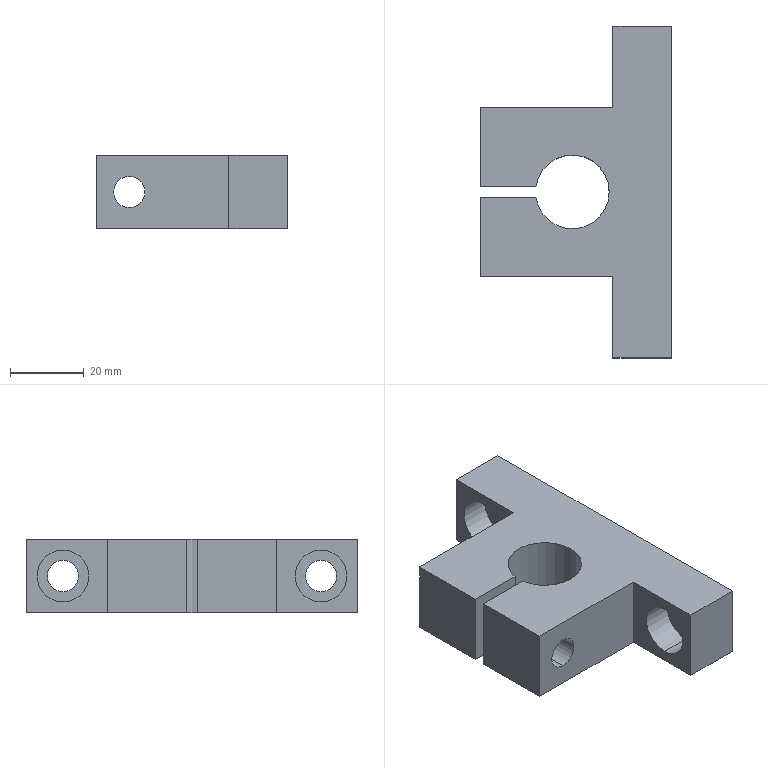Component | SolidWorks | FixedSeat-1 | 1 solid | 31 faces | box 52 x 90 x 20 mm | volume 47991 mm3 | plane 16 | cylinder 15 | commonest cylinder face diameters 8.5 x8 14 x6 20 x1
STEP:
#1=CARTESIAN_POINT('',(-0.4331,19.528,-13.76));
#2=VERTEX_POINT('',#1);
#3=CARTESIAN_POINT('',(-0.4331,19.528,-13.209));
#4=VERTEX_POINT('',#3);
#5=CARTESIAN_POINT('',(-0.4331,19.528,-13.484));
#6=DIRECTION('',(-1.,0.,0.));
#7=DIRECTION('',(0.,0.,1.));
#8=AXIS2_PLACEMENT_3D('',#5,#6,#7);
#9=CIRCLE('',#8,0.2756);
#10=EDGE_CURVE('',#2,#4,#9,.T.);
#11=ORIENTED_EDGE('',*,*,#10,.F.);
#12=CARTESIAN_POINT('',(-0.748,19.528,-13.76));
#13=VERTEX_POINT('',#12);
#14=CARTESIAN_POINT('',(-0.748,19.528,-13.76));
#15=DIRECTION('',(-1.,0.,0.));
#16=VECTOR('',#15,39.37);
#17=LINE('',#14,#16);
#18=EDGE_CURVE('',#2,#13,#17,.T.);
#19=ORIENTED_EDGE('',*,*,#18,.T.);
#20=CARTESIAN_POINT('',(-0.748,19.528,-13.209));
#21=VERTEX_POINT('',#20);
#22=CARTESIAN_POINT('',(-0.748,19.528,-13.484));
#23=DIRECTION('',(-1.,0.,0.));
#24=DIRECTION('',(0.,0.,1.));
#25=AXIS2_PLACEMENT_3D('',#22,#23,#24);
#26=CIRCLE('',#25,0.2756);
#27=EDGE_CURVE('',#13,#21,#26,.T.);
#28=ORIENTED_EDGE('',*,*,#27,.T.);
#29=CARTESIAN_POINT('',(-0.748,19.528,-13.209));
#30=DIRECTION('',(-1.,0.,0.));
#31=VECTOR('',#30,39.37);
#32=LINE('',#29,#31);
#33=EDGE_CURVE('',#4,#21,#32,.T.);
#34=ORIENTED_EDGE('',*,*,#33,.F.);
#35=EDGE_LOOP('',(#11,#19,#28,#34));
#36=FACE_OUTER_BOUND('',#35,.T.);
#37=CARTESIAN_POINT('',(-0.748,19.528,-13.484));
#38=DIRECTION('',(-1.,0.,0.));
#39=DIRECTION('',(0.,0.,1.));
#40=AXIS2_PLACEMENT_3D('',#37,#38,#39);
#41=CYLINDRICAL_SURFACE('',#40,0.2756);
#42=ADVANCED_FACE('',(#36),#41,.F.);
#43=CARTESIAN_POINT('',(-0.1181,19.528,-13.652));
#44=VERTEX_POINT('',#43);
#45=CARTESIAN_POINT('',(-0.1181,19.528,-13.317));
#46=VERTEX_POINT('',#45);
#47=CARTESIAN_POINT('',(-0.1181,19.528,-13.484));
#48=DIRECTION('',(-1.,0.,0.));
#49=DIRECTION('',(0.,0.,1.));
#50=AXIS2_PLACEMENT_3D('',#47,#48,#49);
#51=CIRCLE('',#50,0.1673);
#52=EDGE_CURVE('',#44,#46,#51,.T.);
#53=ORIENTED_EDGE('',*,*,#52,.F.);
#54=CARTESIAN_POINT('',(-0.4331,19.528,-13.652));
#55=VERTEX_POINT('',#54);
#56=CARTESIAN_POINT('',(-0.748,19.528,-13.652));
#57=DIRECTION('',(-1.,0.,0.));
#58=VECTOR('',#57,39.37);
#59=LINE('',#56,#58);
#60=EDGE_CURVE('',#44,#55,#59,.T.);
#61=ORIENTED_EDGE('',*,*,#60,.T.);
#62=CARTESIAN_POINT('',(-0.4331,19.528,-13.317));
#63=VERTEX_POINT('',#62);
#64=CARTESIAN_POINT('',(-0.4331,19.528,-13.484));
#65=DIRECTION('',(-1.,0.,0.));
#66=DIRECTION('',(0.,0.,1.));
#67=AXIS2_PLACEMENT_3D('',#64,#65,#66);
#68=CIRCLE('',#67,0.1673);
#69=EDGE_CURVE('',#55,#63,#68,.T.);
#70=ORIENTED_EDGE('',*,*,#69,.T.);
#71=CARTESIAN_POINT('',(-0.748,19.528,-13.317));
#72=DIRECTION('',(-1.,0.,0.));
#73=VECTOR('',#72,39.37);
#74=LINE('',#71,#73);
#75=EDGE_CURVE('',#46,#63,#74,.T.);
#76=ORIENTED_EDGE('',*,*,#75,.F.);
#77=EDGE_LOOP('',(#53,#61,#70,#76));
#78=FACE_OUTER_BOUND('',#77,.T.);
#79=CARTESIAN_POINT('',(-0.748,19.528,-13.484));
#80=DIRECTION('',(-1.,0.,0.));
#81=DIRECTION('',(0.,0.,1.));
#82=AXIS2_PLACEMENT_3D('',#79,#80,#81);
#83=CYLINDRICAL_SURFACE('',#82,0.1673);
#84=ADVANCED_FACE('',(#78),#83,.F.);
#85=CARTESIAN_POINT('',(-0.4331,16.772,-13.76));
#86=VERTEX_POINT('',#85);
#87=CARTESIAN_POINT('',(-0.4331,16.772,-13.209));
#88=VERTEX_POINT('',#87);
#89=CARTESIAN_POINT('',(-0.4331,16.772,-13.484));
#90=DIRECTION('',(-1.,0.,0.));
#91=DIRECTION('',(0.,0.,1.));
#92=AXIS2_PLACEMENT_3D('',#89,#90,#91);
#93=CIRCLE('',#92,0.2756);
#94=EDGE_CURVE('',#86,#88,#93,.T.);
#95=ORIENTED_EDGE('',*,*,#94,.F.);
#96=CARTESIAN_POINT('',(-0.748,16.772,-13.76));
#97=VERTEX_POINT('',#96);
#98=CARTESIAN_POINT('',(-0.748,16.772,-13.76));
#99=DIRECTION('',(-1.,0.,0.));
#100=VECTOR('',#99,39.37);
#101=LINE('',#98,#100);
#102=EDGE_CURVE('',#86,#97,#101,.T.);
#103=ORIENTED_EDGE('',*,*,#102,.T.);
#104=CARTESIAN_POINT('',(-0.748,16.772,-13.209));
#105=VERTEX_POINT('',#104);
#106=CARTESIAN_POINT('',(-0.748,16.772,-13.484));
#107=DIRECTION('',(-1.,0.,0.));
#108=DIRECTION('',(0.,0.,1.));
#109=AXIS2_PLACEMENT_3D('',#106,#107,#108);
#110=CIRCLE('',#109,0.2756);
#111=EDGE_CURVE('',#97,#105,#110,.T.);
#112=ORIENTED_EDGE('',*,*,#111,.T.);
#113=CARTESIAN_POINT('',(-0.748,16.772,-13.209));
#114=DIRECTION('',(-1.,0.,0.));
#115=VECTOR('',#114,39.37);
#116=LINE('',#113,#115);
#117=EDGE_CURVE('',#88,#105,#116,.T.);
#118=ORIENTED_EDGE('',*,*,#117,.F.);
#119=EDGE_LOOP('',(#95,#103,#112,#118));
#120=FACE_OUTER_BOUND('',#119,.T.);
#121=CARTESIAN_POINT('',(-0.748,16.772,-13.484));
#122=DIRECTION('',(-1.,0.,0.));
#123=DIRECTION('',(0.,0.,1.));
#124=AXIS2_PLACEMENT_3D('',#121,#122,#123);
#125=CYLINDRICAL_SURFACE('',#124,0.2756);
#126=ADVANCED_FACE('',(#120),#125,.F.);
#127=CARTESIAN_POINT('',(-0.1181,16.772,-13.652));
#128=VERTEX_POINT('',#127);
#129=CARTESIAN_POINT('',(-0.1181,16.772,-13.317));
#130=VERTEX_POINT('',#129);
#131=CARTESIAN_POINT('',(-0.1181,16.772,-13.484));
#132=DIRECTION('',(-1.,0.,0.));
#133=DIRECTION('',(0.,0.,1.));
#134=AXIS2_PLACEMENT_3D('',#131,#132,#133);
#135=CIRCLE('',#134,0.1673);
#136=EDGE_CURVE('',#128,#130,#135,.T.);
#137=ORIENTED_EDGE('',*,*,#136,.F.);
#138=CARTESIAN_POINT('',(-0.4331,16.772,-13.652));
#139=VERTEX_POINT('',#138);
#140=CARTESIAN_POINT('',(-0.748,16.772,-13.652));
#141=DIRECTION('',(-1.,0.,0.));
#142=VECTOR('',#141,39.37);
#143=LINE('',#140,#142);
#144=EDGE_CURVE('',#128,#139,#143,.T.);
#145=ORIENTED_EDGE('',*,*,#144,.T.);
#146=CARTESIAN_POINT('',(-0.4331,16.772,-13.317));
#147=VERTEX_POINT('',#146);
#148=CARTESIAN_POINT('',(-0.4331,16.772,-13.484));
#149=DIRECTION('',(-1.,0.,0.));
#150=DIRECTION('',(0.,0.,1.));
#151=AXIS2_PLACEMENT_3D('',#148,#149,#150);
#152=CIRCLE('',#151,0.1673);
#153=EDGE_CURVE('',#139,#147,#152,.T.);
#154=ORIENTED_EDGE('',*,*,#153,.T.);
#155=CARTESIAN_POINT('',(-0.748,16.772,-13.317));
#156=DIRECTION('',(-1.,0.,0.));
#157=VECTOR('',#156,39.37);
#158=LINE('',#155,#157);
#159=EDGE_CURVE('',#130,#147,#158,.T.);
#160=ORIENTED_EDGE('',*,*,#159,.F.);
#161=EDGE_LOOP('',(#137,#145,#154,#160));
#162=FACE_OUTER_BOUND('',#161,.T.);
#163=CARTESIAN_POINT('',(-0.748,16.772,-13.484));
#164=DIRECTION('',(-1.,0.,0.));
#165=DIRECTION('',(0.,0.,1.));
#166=AXIS2_PLACEMENT_3D('',#163,#164,#165);
#167=CYLINDRICAL_SURFACE('',#166,0.1673);
#168=ADVANCED_FACE('',(#162),#167,.F.);
#169=CARTESIAN_POINT('',(-1.811,18.677,-13.76));
#170=VERTEX_POINT('',#169);
#171=CARTESIAN_POINT('',(-1.811,18.677,-13.209));
#172=VERTEX_POINT('',#171);
#173=CARTESIAN_POINT('',(-1.811,18.677,-13.484));
#174=DIRECTION('',(0.,1.,0.));
#175=DIRECTION('',(0.,0.,1.));
#176=AXIS2_PLACEMENT_3D('',#173,#174,#175);
#177=CIRCLE('',#176,0.2756);
#178=EDGE_CURVE('',#170,#172,#177,.T.);
#179=ORIENTED_EDGE('',*,*,#178,.F.);
#180=CARTESIAN_POINT('',(-1.811,19.055,-13.76));
#181=VERTEX_POINT('',#180);
#182=CARTESIAN_POINT('',(-1.811,19.055,-13.76));
#183=DIRECTION('',(0.,1.,0.));
#184=VECTOR('',#183,39.37);
#185=LINE('',#182,#184);
#186=EDGE_CURVE('',#170,#181,#185,.T.);
#187=ORIENTED_EDGE('',*,*,#186,.T.);
#188=CARTESIAN_POINT('',(-1.811,19.055,-13.209));
#189=VERTEX_POINT('',#188);
#190=CARTESIAN_POINT('',(-1.811,19.055,-13.484));
#191=DIRECTION('',(0.,1.,0.));
#192=DIRECTION('',(0.,0.,1.));
#193=AXIS2_PLACEMENT_3D('',#190,#191,#192);
#194=CIRCLE('',#193,0.2756);
#195=EDGE_CURVE('',#181,#189,#194,.T.);
#196=ORIENTED_EDGE('',*,*,#195,.T.);
#197=CARTESIAN_POINT('',(-1.811,19.055,-13.209));
#198=DIRECTION('',(0.,1.,0.));
#199=VECTOR('',#198,39.37);
#200=LINE('',#197,#199);
#201=EDGE_CURVE('',#172,#189,#200,.T.);
#202=ORIENTED_EDGE('',*,*,#201,.F.);
#203=EDGE_LOOP('',(#179,#187,#196,#202));
#204=FACE_OUTER_BOUND('',#203,.T.);
#205=CARTESIAN_POINT('',(-1.811,19.055,-13.484));
#206=DIRECTION('',(0.,1.,0.));
#207=DIRECTION('',(0.,0.,1.));
#208=AXIS2_PLACEMENT_3D('',#205,#206,#207);
#209=CYLINDRICAL_SURFACE('',#208,0.2756);
#210=ADVANCED_FACE('',(#204),#209,.F.);
#211=CARTESIAN_POINT('',(-1.811,18.209,-13.652));
#212=VERTEX_POINT('',#211);
#213=CARTESIAN_POINT('',(-1.811,18.209,-13.317));
#214=VERTEX_POINT('',#213);
#215=CARTESIAN_POINT('',(-1.811,18.209,-13.484));
#216=DIRECTION('',(-0.,1.,0.));
#217=DIRECTION('',(-1.,0.,0.));
#218=AXIS2_PLACEMENT_3D('',#215,#216,#217);
#219=CIRCLE('',#218,0.1673);
#220=EDGE_CURVE('',#212,#214,#219,.T.);
#221=ORIENTED_EDGE('',*,*,#220,.F.);
#222=CARTESIAN_POINT('',(-1.811,18.677,-13.652));
#223=VERTEX_POINT('',#222);
#224=CARTESIAN_POINT('',(-1.811,19.055,-13.652));
#225=DIRECTION('',(0.,1.,0.));
#226=VECTOR('',#225,39.37);
#227=LINE('',#224,#226);
#228=EDGE_CURVE('',#212,#223,#227,.T.);
#229=ORIENTED_EDGE('',*,*,#228,.T.);
#230=CARTESIAN_POINT('',(-1.811,18.677,-13.317));
#231=VERTEX_POINT('',#230);
#232=CARTESIAN_POINT('',(-1.811,18.677,-13.484));
#233=DIRECTION('',(0.,1.,0.));
#234=DIRECTION('',(0.,0.,1.));
#235=AXIS2_PLACEMENT_3D('',#232,#233,#234);
#236=CIRCLE('',#235,0.1673);
#237=EDGE_CURVE('',#223,#231,#236,.T.);
#238=ORIENTED_EDGE('',*,*,#237,.T.);
#239=CARTESIAN_POINT('',(-1.811,19.055,-13.317));
#240=DIRECTION('',(0.,1.,0.));
#241=VECTOR('',#240,39.37);
#242=LINE('',#239,#241);
#243=EDGE_CURVE('',#214,#231,#242,.T.);
#244=ORIENTED_EDGE('',*,*,#243,.F.);
#245=EDGE_LOOP('',(#221,#229,#238,#244));
#246=FACE_OUTER_BOUND('',#245,.T.);
#247=CARTESIAN_POINT('',(-1.811,19.055,-13.484));
#248=DIRECTION('',(0.,1.,0.));
#249=DIRECTION('',(0.,0.,1.));
#250=AXIS2_PLACEMENT_3D('',#247,#248,#249);
#251=CYLINDRICAL_SURFACE('',#250,0.1673);
#252=ADVANCED_FACE('',(#246),#251,.F.);
#253=CARTESIAN_POINT('',(-1.811,17.244,-13.652));
#254=VERTEX_POINT('',#253);
#255=CARTESIAN_POINT('',(-1.811,17.244,-13.317));
#256=VERTEX_POINT('',#255);
#257=CARTESIAN_POINT('',(-1.811,17.244,-13.484));
#258=DIRECTION('',(0.,1.,0.));
#259=DIRECTION('',(0.,0.,1.));
#260=AXIS2_PLACEMENT_3D('',#257,#258,#259);
#261=CIRCLE('',#260,0.1673);
#262=EDGE_CURVE('',#254,#256,#261,.T.);
#263=ORIENTED_EDGE('',*,*,#262,.F.);
#264=CARTESIAN_POINT('',(-1.811,18.091,-13.652));
#265=VERTEX_POINT('',#264);
#266=CARTESIAN_POINT('',(-1.811,19.055,-13.652));
#267=DIRECTION('',(0.,1.,0.));
#268=VECTOR('',#267,39.37);
#269=LINE('',#266,#268);
#270=EDGE_CURVE('',#254,#265,#269,.T.);
#271=ORIENTED_EDGE('',*,*,#270,.T.);
#272=CARTESIAN_POINT('',(-1.811,18.091,-13.317));
#273=VERTEX_POINT('',#272);
#274=CARTESIAN_POINT('',(-1.811,18.091,-13.484));
#275=DIRECTION('',(0.,-1.,0.));
#276=DIRECTION('',(1.,0.,0.));
#277=AXIS2_PLACEMENT_3D('',#274,#275,#276);
#278=CIRCLE('',#277,0.1673);
#279=EDGE_CURVE('',#273,#265,#278,.T.);
#280=ORIENTED_EDGE('',*,*,#279,.F.);
#281=CARTESIAN_POINT('',(-1.811,19.055,-13.317));
#282=DIRECTION('',(0.,1.,0.));
#283=VECTOR('',#282,39.37);
#284=LINE('',#281,#283);
#285=EDGE_CURVE('',#256,#273,#284,.T.);
#286=ORIENTED_EDGE('',*,*,#285,.F.);
#287=EDGE_LOOP('',(#263,#271,#280,#286));
#288=FACE_OUTER_BOUND('',#287,.T.);
#289=CARTESIAN_POINT('',(-1.811,19.055,-13.484));
#290=DIRECTION('',(0.,1.,0.));
#291=DIRECTION('',(0.,0.,1.));
#292=AXIS2_PLACEMENT_3D('',#289,#290,#291);
#293=CYLINDRICAL_SURFACE('',#292,0.1673);
#294=ADVANCED_FACE('',(#288),#293,.F.);
#295=CARTESIAN_POINT('',(-2.165,19.055,-13.878));
#296=VERTEX_POINT('',#295);
#297=CARTESIAN_POINT('',(-2.165,19.055,-13.091));
#298=VERTEX_POINT('',#297);
#299=CARTESIAN_POINT('',(-2.165,19.055,-13.878));
#300=DIRECTION('',(0.,0.,1.));
#301=VECTOR('',#300,39.37);
#302=LINE('',#299,#301);
#303=EDGE_CURVE('',#296,#298,#302,.T.);
#304=ORIENTED_EDGE('',*,*,#303,.F.);
#305=CARTESIAN_POINT('',(-2.165,18.209,-13.878));
#306=VERTEX_POINT('',#305);
#307=CARTESIAN_POINT('',(-2.165,16.378,-13.878));
#308=DIRECTION('',(0.,1.,0.));
#309=VECTOR('',#308,39.37);
#310=LINE('',#307,#309);
#311=EDGE_CURVE('',#306,#296,#310,.T.);
#312=ORIENTED_EDGE('',*,*,#311,.F.);
#313=CARTESIAN_POINT('',(-2.165,18.209,-13.091));
#314=VERTEX_POINT('',#313);
#315=CARTESIAN_POINT('',(-2.165,18.209,-13.878));
#316=DIRECTION('',(0.,0.,1.));
#317=VECTOR('',#316,39.37);
#318=LINE('',#315,#317);
#319=EDGE_CURVE('',#306,#314,#318,.T.);
#320=ORIENTED_EDGE('',*,*,#319,.T.);
#321=CARTESIAN_POINT('',(-2.165,16.378,-13.091));
#322=DIRECTION('',(0.,1.,0.));
#323=VECTOR('',#322,39.37);
#324=LINE('',#321,#323);
#325=EDGE_CURVE('',#314,#298,#324,.T.);
#326=ORIENTED_EDGE('',*,*,#325,.T.);
#327=EDGE_LOOP('',(#304,#312,#320,#326));
#328=FACE_OUTER_BOUND('',#327,.T.);
#329=CARTESIAN_POINT('',(-2.165,16.378,-13.091));
#330=DIRECTION('',(-1.,0.,0.));
#331=DIRECTION('',(0.,0.,1.));
#332=AXIS2_PLACEMENT_3D('',#329,#330,#331);
#333=PLANE('',#332);
#334=ADVANCED_FACE('',(#328),#333,.T.);
#335=CARTESIAN_POINT('',(-0.748,16.378,-13.878));
#336=VERTEX_POINT('',#335);
#337=CARTESIAN_POINT('',(-0.748,16.378,-13.091));
#338=VERTEX_POINT('',#337);
#339=CARTESIAN_POINT('',(-0.748,16.378,-13.878));
#340=DIRECTION('',(0.,0.,1.));
#341=VECTOR('',#340,39.37);
#342=LINE('',#339,#341);
#343=EDGE_CURVE('',#336,#338,#342,.T.);
#344=ORIENTED_EDGE('',*,*,#343,.F.);
#345=CARTESIAN_POINT('',(-0.1181,16.378,-13.878));
#346=VERTEX_POINT('',#345);
#347=CARTESIAN_POINT('',(-0.1181,16.378,-13.878));
#348=DIRECTION('',(-1.,0.,0.));
#349=VECTOR('',#348,39.37);
#350=LINE('',#347,#349);
#351=EDGE_CURVE('',#346,#336,#350,.T.);
#352=ORIENTED_EDGE('',*,*,#351,.F.);
#353=CARTESIAN_POINT('',(-0.1181,16.378,-13.091));
#354=VERTEX_POINT('',#353);
#355=CARTESIAN_POINT('',(-0.1181,16.378,-13.091));
#356=DIRECTION('',(0.,0.,-1.));
#357=VECTOR('',#356,39.37);
#358=LINE('',#355,#357);
#359=EDGE_CURVE('',#354,#346,#358,.T.);
#360=ORIENTED_EDGE('',*,*,#359,.F.);
#361=CARTESIAN_POINT('',(-0.1181,16.378,-13.091));
#362=DIRECTION('',(-1.,0.,0.));
#363=VECTOR('',#362,39.37);
#364=LINE('',#361,#363);
#365=EDGE_CURVE('',#354,#338,#364,.T.);
#366=ORIENTED_EDGE('',*,*,#365,.T.);
#367=EDGE_LOOP('',(#344,#352,#360,#366));
#368=FACE_OUTER_BOUND('',#367,.T.);
#369=CARTESIAN_POINT('',(-0.1181,16.378,-13.091));
#370=DIRECTION('',(0.,-1.,0.));
#371=DIRECTION('',(0.,0.,-1.));
#372=AXIS2_PLACEMENT_3D('',#369,#370,#371);
#373=PLANE('',#372);
#374=ADVANCED_FACE('',(#368),#373,.T.);
#375=CARTESIAN_POINT('',(-0.1181,19.528,-13.484));
#376=DIRECTION('',(-1.,0.,0.));
#377=DIRECTION('',(0.,0.,1.));
#378=AXIS2_PLACEMENT_3D('',#375,#376,#377);
#379=CIRCLE('',#378,0.1673);
#380=EDGE_CURVE('',#46,#44,#379,.T.);
#381=ORIENTED_EDGE('',*,*,#380,.T.);
#382=ORIENTED_EDGE('',*,*,#52,.T.);
#383=EDGE_LOOP('',(#381,#382));
#384=FACE_BOUND('',#383,.T.);
#385=CARTESIAN_POINT('',(-0.1181,16.772,-13.484));
#386=DIRECTION('',(-1.,0.,0.));
#387=DIRECTION('',(0.,0.,1.));
#388=AXIS2_PLACEMENT_3D('',#385,#386,#387);
#389=CIRCLE('',#388,0.1673);
#390=EDGE_CURVE('',#130,#128,#389,.T.);
#391=ORIENTED_EDGE('',*,*,#390,.T.);
#392=ORIENTED_EDGE('',*,*,#136,.T.);
#393=EDGE_LOOP('',(#391,#392));
#394=FACE_BOUND('',#393,.T.);
#395=CARTESIAN_POINT('',(-0.1181,19.921,-13.878));
#396=VERTEX_POINT('',#395);
#397=CARTESIAN_POINT('',(-0.1181,19.921,-13.878));
#398=DIRECTION('',(0.,-1.,0.));
#399=VECTOR('',#398,39.37);
#400=LINE('',#397,#399);
#401=EDGE_CURVE('',#396,#346,#400,.T.);
#402=ORIENTED_EDGE('',*,*,#401,.F.);
#403=CARTESIAN_POINT('',(-0.1181,19.921,-13.091));
#404=VERTEX_POINT('',#403);
#405=CARTESIAN_POINT('',(-0.1181,19.921,-13.091));
#406=DIRECTION('',(0.,0.,-1.));
#407=VECTOR('',#406,39.37);
#408=LINE('',#405,#407);
#409=EDGE_CURVE('',#404,#396,#408,.T.);
#410=ORIENTED_EDGE('',*,*,#409,.F.);
#411=CARTESIAN_POINT('',(-0.1181,19.921,-13.091));
#412=DIRECTION('',(0.,-1.,0.));
#413=VECTOR('',#412,39.37);
#414=LINE('',#411,#413);
#415=EDGE_CURVE('',#404,#354,#414,.T.);
#416=ORIENTED_EDGE('',*,*,#415,.T.);
#417=ORIENTED_EDGE('',*,*,#359,.T.);
#418=EDGE_LOOP('',(#402,#410,#416,#417));
#419=FACE_OUTER_BOUND('',#418,.T.);
#420=CARTESIAN_POINT('',(-0.1181,19.921,-13.091));
#421=DIRECTION('',(1.,0.,0.));
#422=DIRECTION('',(-0.,1.,0.));
#423=AXIS2_PLACEMENT_3D('',#420,#421,#422);
#424=PLANE('',#423);
#425=ADVANCED_FACE('',(#384,#394,#419),#424,.T.);
#426=CARTESIAN_POINT('',(-0.748,19.921,-13.878));
#427=VERTEX_POINT('',#426);
#428=CARTESIAN_POINT('',(-0.748,19.921,-13.091));
#429=VERTEX_POINT('',#428);
#430=CARTESIAN_POINT('',(-0.748,19.921,-13.878));
#431=DIRECTION('',(0.,0.,1.));
#432=VECTOR('',#431,39.37);
#433=LINE('',#430,#432);
#434=EDGE_CURVE('',#427,#429,#433,.T.);
#435=ORIENTED_EDGE('',*,*,#434,.T.);
#436=CARTESIAN_POINT('',(-2.165,19.921,-13.091));
#437=DIRECTION('',(1.,0.,0.));
#438=VECTOR('',#437,39.37);
#439=LINE('',#436,#438);
#440=EDGE_CURVE('',#429,#404,#439,.T.);
#441=ORIENTED_EDGE('',*,*,#440,.T.);
#442=ORIENTED_EDGE('',*,*,#409,.T.);
#443=CARTESIAN_POINT('',(-2.165,19.921,-13.878));
#444=DIRECTION('',(1.,0.,0.));
#445=VECTOR('',#444,39.37);
#446=LINE('',#443,#445);
#447=EDGE_CURVE('',#427,#396,#446,.T.);
#448=ORIENTED_EDGE('',*,*,#447,.F.);
#449=EDGE_LOOP('',(#435,#441,#442,#448));
#450=FACE_OUTER_BOUND('',#449,.T.);
#451=CARTESIAN_POINT('',(-2.165,19.921,-13.091));
#452=DIRECTION('',(0.,1.,0.));
#453=DIRECTION('',(0.,0.,1.));
#454=AXIS2_PLACEMENT_3D('',#451,#452,#453);
#455=PLANE('',#454);
#456=ADVANCED_FACE('',(#450),#455,.T.);
#457=CARTESIAN_POINT('',(-2.165,17.244,-13.878));
#458=VERTEX_POINT('',#457);
#459=CARTESIAN_POINT('',(-2.165,17.244,-13.091));
#460=VERTEX_POINT('',#459);
#461=CARTESIAN_POINT('',(-2.165,17.244,-13.878));
#462=DIRECTION('',(0.,0.,1.));
#463=VECTOR('',#462,39.37);
#464=LINE('',#461,#463);
#465=EDGE_CURVE('',#458,#460,#464,.T.);
#466=ORIENTED_EDGE('',*,*,#465,.T.);
#467=CARTESIAN_POINT('',(-2.165,18.091,-13.091));
#468=VERTEX_POINT('',#467);
#469=CARTESIAN_POINT('',(-2.165,16.378,-13.091));
#470=DIRECTION('',(0.,1.,0.));
#471=VECTOR('',#470,39.37);
#472=LINE('',#469,#471);
#473=EDGE_CURVE('',#460,#468,#472,.T.);
#474=ORIENTED_EDGE('',*,*,#473,.T.);
#475=CARTESIAN_POINT('',(-2.165,18.091,-13.878));
#476=VERTEX_POINT('',#475);
#477=CARTESIAN_POINT('',(-2.165,18.091,-13.878));
#478=DIRECTION('',(0.,0.,1.));
#479=VECTOR('',#478,39.37);
#480=LINE('',#477,#479);
#481=EDGE_CURVE('',#476,#468,#480,.T.);
#482=ORIENTED_EDGE('',*,*,#481,.F.);
#483=CARTESIAN_POINT('',(-2.165,16.378,-13.878));
#484=DIRECTION('',(0.,1.,0.));
#485=VECTOR('',#484,39.37);
#486=LINE('',#483,#485);
#487=EDGE_CURVE('',#458,#476,#486,.T.);
#488=ORIENTED_EDGE('',*,*,#487,.F.);
#489=EDGE_LOOP('',(#466,#474,#482,#488));
#490=FACE_OUTER_BOUND('',#489,.T.);
#491=CARTESIAN_POINT('',(-2.165,16.378,-13.091));
#492=DIRECTION('',(-1.,0.,0.));
#493=DIRECTION('',(0.,0.,1.));
#494=AXIS2_PLACEMENT_3D('',#491,#492,#493);
#495=PLANE('',#494);
#496=ADVANCED_FACE('',(#490),#495,.T.);
#497=CARTESIAN_POINT('',(-1.57,18.209,-13.091));
#498=VERTEX_POINT('',#497);
#499=CARTESIAN_POINT('',(-1.57,18.209,-13.091));
#500=DIRECTION('',(-1.,-0.,0.));
#501=VECTOR('',#500,39.37);
#502=LINE('',#499,#501);
#503=EDGE_CURVE('',#498,#314,#502,.T.);
#504=ORIENTED_EDGE('',*,*,#503,.F.);
#505=CARTESIAN_POINT('',(-1.57,18.091,-13.091));
#506=VERTEX_POINT('',#505);
#507=CARTESIAN_POINT('',(-1.181,18.15,-13.091));
#508=DIRECTION('',(0.,0.,-1.));
#509=DIRECTION('',(-1.,0.,0.));
#510=AXIS2_PLACEMENT_3D('',#507,#508,#509);
#511=CIRCLE('',#510,0.3937);
#512=EDGE_CURVE('',#498,#506,#511,.T.);
#513=ORIENTED_EDGE('',*,*,#512,.T.);
#514=CARTESIAN_POINT('',(-2.165,18.091,-13.091));
#515=DIRECTION('',(1.,0.,0.));
#516=VECTOR('',#515,39.37);
#517=LINE('',#514,#516);
#518=EDGE_CURVE('',#468,#506,#517,.T.);
#519=ORIENTED_EDGE('',*,*,#518,.F.);
#520=ORIENTED_EDGE('',*,*,#473,.F.);
#521=CARTESIAN_POINT('',(-0.748,17.244,-13.091));
#522=VERTEX_POINT('',#521);
#523=CARTESIAN_POINT('',(-0.748,17.244,-13.091));
#524=DIRECTION('',(-1.,0.,0.));
#525=VECTOR('',#524,39.37);
#526=LINE('',#523,#525);
#527=EDGE_CURVE('',#522,#460,#526,.T.);
#528=ORIENTED_EDGE('',*,*,#527,.F.);
#529=CARTESIAN_POINT('',(-0.748,16.378,-13.091));
#530=DIRECTION('',(0.,1.,0.));
#531=VECTOR('',#530,39.37);
#532=LINE('',#529,#531);
#533=EDGE_CURVE('',#338,#522,#532,.T.);
#534=ORIENTED_EDGE('',*,*,#533,.F.);
#535=ORIENTED_EDGE('',*,*,#365,.F.);
#536=ORIENTED_EDGE('',*,*,#415,.F.);
#537=ORIENTED_EDGE('',*,*,#440,.F.);
#538=CARTESIAN_POINT('',(-0.748,19.055,-13.091));
#539=VERTEX_POINT('',#538);
#540=CARTESIAN_POINT('',(-0.748,19.055,-13.091));
#541=DIRECTION('',(0.,1.,0.));
#542=VECTOR('',#541,39.37);
#543=LINE('',#540,#542);
#544=EDGE_CURVE('',#539,#429,#543,.T.);
#545=ORIENTED_EDGE('',*,*,#544,.F.);
#546=CARTESIAN_POINT('',(-2.165,19.055,-13.091));
#547=DIRECTION('',(1.,0.,0.));
#548=VECTOR('',#547,39.37);
#549=LINE('',#546,#548);
#550=EDGE_CURVE('',#298,#539,#549,.T.);
#551=ORIENTED_EDGE('',*,*,#550,.F.);
#552=ORIENTED_EDGE('',*,*,#325,.F.);
#553=EDGE_LOOP('',(#504,#513,#519,#520,#528,#534,#535,#536,#537,#545,#551,#552));
#554=FACE_OUTER_BOUND('',#553,.T.);
#555=CARTESIAN_POINT('',(-0.1181,18.15,-13.091));
#556=DIRECTION('',(0.,0.,-1.));
#557=DIRECTION('',(-1.,0.,0.));
#558=AXIS2_PLACEMENT_3D('',#555,#556,#557);
#559=PLANE('',#558);
#560=ADVANCED_FACE('',(#554),#559,.F.);
#561=CARTESIAN_POINT('',(-1.57,18.209,-13.878));
#562=VERTEX_POINT('',#561);
#563=CARTESIAN_POINT('',(-1.57,18.091,-13.878));
#564=VERTEX_POINT('',#563);
#565=CARTESIAN_POINT('',(-1.181,18.15,-13.878));
#566=DIRECTION('',(0.,0.,-1.));
#567=DIRECTION('',(-1.,0.,0.));
#568=AXIS2_PLACEMENT_3D('',#565,#566,#567);
#569=CIRCLE('',#568,0.3937);
#570=EDGE_CURVE('',#562,#564,#569,.T.);
#571=ORIENTED_EDGE('',*,*,#570,.F.);
#572=CARTESIAN_POINT('',(-1.57,18.209,-13.878));
#573=DIRECTION('',(-1.,-0.,0.));
#574=VECTOR('',#573,39.37);
#575=LINE('',#572,#574);
#576=EDGE_CURVE('',#562,#306,#575,.T.);
#577=ORIENTED_EDGE('',*,*,#576,.T.);
#578=ORIENTED_EDGE('',*,*,#311,.T.);
#579=CARTESIAN_POINT('',(-0.748,19.055,-13.878));
#580=VERTEX_POINT('',#579);
#581=CARTESIAN_POINT('',(-2.165,19.055,-13.878));
#582=DIRECTION('',(1.,0.,0.));
#583=VECTOR('',#582,39.37);
#584=LINE('',#581,#583);
#585=EDGE_CURVE('',#296,#580,#584,.T.);
#586=ORIENTED_EDGE('',*,*,#585,.T.);
#587=CARTESIAN_POINT('',(-0.748,19.055,-13.878));
#588=DIRECTION('',(0.,1.,0.));
#589=VECTOR('',#588,39.37);
#590=LINE('',#587,#589);
#591=EDGE_CURVE('',#580,#427,#590,.T.);
#592=ORIENTED_EDGE('',*,*,#591,.T.);
#593=ORIENTED_EDGE('',*,*,#447,.T.);
#594=ORIENTED_EDGE('',*,*,#401,.T.);
#595=ORIENTED_EDGE('',*,*,#351,.T.);
#596=CARTESIAN_POINT('',(-0.748,17.244,-13.878));
#597=VERTEX_POINT('',#596);
#598=CARTESIAN_POINT('',(-0.748,16.378,-13.878));
#599=DIRECTION('',(0.,1.,0.));
#600=VECTOR('',#599,39.37);
#601=LINE('',#598,#600);
#602=EDGE_CURVE('',#336,#597,#601,.T.);
#603=ORIENTED_EDGE('',*,*,#602,.T.);
#604=CARTESIAN_POINT('',(-0.748,17.244,-13.878));
#605=DIRECTION('',(-1.,0.,0.));
#606=VECTOR('',#605,39.37);
#607=LINE('',#604,#606);
#608=EDGE_CURVE('',#597,#458,#607,.T.);
#609=ORIENTED_EDGE('',*,*,#608,.T.);
#610=ORIENTED_EDGE('',*,*,#487,.T.);
#611=CARTESIAN_POINT('',(-2.165,18.091,-13.878));
#612=DIRECTION('',(1.,0.,0.));
#613=VECTOR('',#612,39.37);
#614=LINE('',#611,#613);
#615=EDGE_CURVE('',#476,#564,#614,.T.);
#616=ORIENTED_EDGE('',*,*,#615,.T.);
#617=EDGE_LOOP('',(#571,#577,#578,#586,#592,#593,#594,#595,#603,#609,#610,#616));
#618=FACE_OUTER_BOUND('',#617,.T.);
#619=CARTESIAN_POINT('',(-0.1181,18.15,-13.878));
#620=DIRECTION('',(0.,0.,-1.));
#621=DIRECTION('',(-1.,0.,0.));
#622=AXIS2_PLACEMENT_3D('',#619,#620,#621);
#623=PLANE('',#622);
#624=ADVANCED_FACE('',(#618),#623,.T.);
#625=CARTESIAN_POINT('',(-1.811,18.209,-13.484));
#626=DIRECTION('',(-0.,1.,0.));
#627=DIRECTION('',(-1.,0.,0.));
#628=AXIS2_PLACEMENT_3D('',#625,#626,#627);
#629=CIRCLE('',#628,0.1673);
#630=EDGE_CURVE('',#214,#212,#629,.T.);
#631=ORIENTED_EDGE('',*,*,#630,.T.);
#632=ORIENTED_EDGE('',*,*,#220,.T.);
#633=EDGE_LOOP('',(#631,#632));
#634=FACE_BOUND('',#633,.T.);
#635=ORIENTED_EDGE('',*,*,#503,.T.);
#636=ORIENTED_EDGE('',*,*,#319,.F.);
#637=ORIENTED_EDGE('',*,*,#576,.F.);
#638=CARTESIAN_POINT('',(-1.57,18.209,-13.878));
#639=DIRECTION('',(0.,0.,1.));
#640=VECTOR('',#639,39.37);
#641=LINE('',#638,#640);
#642=EDGE_CURVE('',#562,#498,#641,.T.);
#643=ORIENTED_EDGE('',*,*,#642,.T.);
#644=EDGE_LOOP('',(#635,#636,#637,#643));
#645=FACE_OUTER_BOUND('',#644,.T.);
#646=CARTESIAN_POINT('',(-1.57,18.209,-13.878));
#647=DIRECTION('',(-0.,1.,0.));
#648=DIRECTION('',(-1.,-0.,0.));
#649=AXIS2_PLACEMENT_3D('',#646,#647,#648);
#650=PLANE('',#649);
#651=ADVANCED_FACE('',(#634,#645),#650,.F.);
#652=ORIENTED_EDGE('',*,*,#279,.T.);
#653=CARTESIAN_POINT('',(-1.811,18.091,-13.484));
#654=DIRECTION('',(0.,-1.,0.));
#655=DIRECTION('',(1.,0.,0.));
#656=AXIS2_PLACEMENT_3D('',#653,#654,#655);
#657=CIRCLE('',#656,0.1673);
#658=EDGE_CURVE('',#265,#273,#657,.T.);
#659=ORIENTED_EDGE('',*,*,#658,.T.);
#660=EDGE_LOOP('',(#652,#659));
#661=FACE_BOUND('',#660,.T.);
#662=ORIENTED_EDGE('',*,*,#518,.T.);
#663=CARTESIAN_POINT('',(-1.57,18.091,-13.878));
#664=DIRECTION('',(0.,0.,1.));
#665=VECTOR('',#664,39.37);
#666=LINE('',#663,#665);
#667=EDGE_CURVE('',#564,#506,#666,.T.);
#668=ORIENTED_EDGE('',*,*,#667,.F.);
#669=ORIENTED_EDGE('',*,*,#615,.F.);
#670=ORIENTED_EDGE('',*,*,#481,.T.);
#671=EDGE_LOOP('',(#662,#668,#669,#670));
#672=FACE_OUTER_BOUND('',#671,.T.);
#673=CARTESIAN_POINT('',(-2.165,18.091,-13.878));
#674=DIRECTION('',(0.,-1.,0.));
#675=DIRECTION('',(1.,0.,0.));
#676=AXIS2_PLACEMENT_3D('',#673,#674,#675);
#677=PLANE('',#676);
#678=ADVANCED_FACE('',(#661,#672),#677,.F.);
#679=CARTESIAN_POINT('',(-0.748,19.528,-13.484));
#680=DIRECTION('',(-1.,0.,0.));
#681=DIRECTION('',(0.,0.,1.));
#682=AXIS2_PLACEMENT_3D('',#679,#680,#681);
#683=CIRCLE('',#682,0.2756);
#684=EDGE_CURVE('',#21,#13,#683,.T.);
#685=ORIENTED_EDGE('',*,*,#684,.F.);
#686=ORIENTED_EDGE('',*,*,#27,.F.);
#687=EDGE_LOOP('',(#685,#686));
#688=FACE_BOUND('',#687,.T.);
#689=ORIENTED_EDGE('',*,*,#544,.T.);
#690=ORIENTED_EDGE('',*,*,#434,.F.);
#691=ORIENTED_EDGE('',*,*,#591,.F.);
#692=CARTESIAN_POINT('',(-0.748,19.055,-13.878));
#693=DIRECTION('',(0.,0.,1.));
#694=VECTOR('',#693,39.37);
#695=LINE('',#692,#694);
#696=EDGE_CURVE('',#580,#539,#695,.T.);
#697=ORIENTED_EDGE('',*,*,#696,.T.);
#698=EDGE_LOOP('',(#689,#690,#691,#697));
#699=FACE_OUTER_BOUND('',#698,.T.);
#700=CARTESIAN_POINT('',(-0.748,19.055,-13.878));
#701=DIRECTION('',(1.,0.,0.));
#702=DIRECTION('',(0.,0.,-1.));
#703=AXIS2_PLACEMENT_3D('',#700,#701,#702);
#704=PLANE('',#703);
#705=ADVANCED_FACE('',(#688,#699),#704,.F.);
#706=CARTESIAN_POINT('',(-1.811,19.055,-13.484));
#707=DIRECTION('',(0.,1.,0.));
#708=DIRECTION('',(0.,0.,1.));
#709=AXIS2_PLACEMENT_3D('',#706,#707,#708);
#710=CIRCLE('',#709,0.2756);
#711=EDGE_CURVE('',#189,#181,#710,.T.);
#712=ORIENTED_EDGE('',*,*,#711,.F.);
#713=ORIENTED_EDGE('',*,*,#195,.F.);
#714=EDGE_LOOP('',(#712,#713));
#715=FACE_BOUND('',#714,.T.);
#716=ORIENTED_EDGE('',*,*,#550,.T.);
#717=ORIENTED_EDGE('',*,*,#696,.F.);
#718=ORIENTED_EDGE('',*,*,#585,.F.);
#719=ORIENTED_EDGE('',*,*,#303,.T.);
#720=EDGE_LOOP('',(#716,#717,#718,#719));
#721=FACE_OUTER_BOUND('',#720,.T.);
#722=CARTESIAN_POINT('',(-2.165,19.055,-13.878));
#723=DIRECTION('',(0.,-1.,0.));
#724=DIRECTION('',(0.,0.,-1.));
#725=AXIS2_PLACEMENT_3D('',#722,#723,#724);
#726=PLANE('',#725);
#727=ADVANCED_FACE('',(#715,#721),#726,.F.);
#728=CARTESIAN_POINT('',(-1.811,17.244,-13.484));
#729=DIRECTION('',(0.,1.,0.));
#730=DIRECTION('',(0.,0.,1.));
#731=AXIS2_PLACEMENT_3D('',#728,#729,#730);
#732=CIRCLE('',#731,0.1673);
#733=EDGE_CURVE('',#256,#254,#732,.T.);
#734=ORIENTED_EDGE('',*,*,#733,.T.);
#735=ORIENTED_EDGE('',*,*,#262,.T.);
#736=EDGE_LOOP('',(#734,#735));
#737=FACE_BOUND('',#736,.T.);
#738=ORIENTED_EDGE('',*,*,#527,.T.);
#739=ORIENTED_EDGE('',*,*,#465,.F.);
#740=ORIENTED_EDGE('',*,*,#608,.F.);
#741=CARTESIAN_POINT('',(-0.748,17.244,-13.878));
#742=DIRECTION('',(0.,0.,1.));
#743=VECTOR('',#742,39.37);
#744=LINE('',#741,#743);
#745=EDGE_CURVE('',#597,#522,#744,.T.);
#746=ORIENTED_EDGE('',*,*,#745,.T.);
#747=EDGE_LOOP('',(#738,#739,#740,#746));
#748=FACE_OUTER_BOUND('',#747,.T.);
#749=CARTESIAN_POINT('',(-0.748,17.244,-13.878));
#750=DIRECTION('',(0.,1.,0.));
#751=DIRECTION('',(0.,0.,1.));
#752=AXIS2_PLACEMENT_3D('',#749,#750,#751);
#753=PLANE('',#752);
#754=ADVANCED_FACE('',(#737,#748),#753,.F.);
#755=CARTESIAN_POINT('',(-0.748,16.772,-13.484));
#756=DIRECTION('',(-1.,0.,0.));
#757=DIRECTION('',(0.,0.,1.));
#758=AXIS2_PLACEMENT_3D('',#755,#756,#757);
#759=CIRCLE('',#758,0.2756);
#760=EDGE_CURVE('',#105,#97,#759,.T.);
#761=ORIENTED_EDGE('',*,*,#760,.F.);
#762=ORIENTED_EDGE('',*,*,#111,.F.);
#763=EDGE_LOOP('',(#761,#762));
#764=FACE_BOUND('',#763,.T.);
#765=ORIENTED_EDGE('',*,*,#533,.T.);
#766=ORIENTED_EDGE('',*,*,#745,.F.);
#767=ORIENTED_EDGE('',*,*,#602,.F.);
#768=ORIENTED_EDGE('',*,*,#343,.T.);
#769=EDGE_LOOP('',(#765,#766,#767,#768));
#770=FACE_OUTER_BOUND('',#769,.T.);
#771=CARTESIAN_POINT('',(-0.748,16.378,-13.878));
#772=DIRECTION('',(1.,0.,0.));
#773=DIRECTION('',(0.,0.,-1.));
#774=AXIS2_PLACEMENT_3D('',#771,#772,#773);
#775=PLANE('',#774);
#776=ADVANCED_FACE('',(#764,#770),#775,.F.);
#777=ORIENTED_EDGE('',*,*,#570,.T.);
#778=ORIENTED_EDGE('',*,*,#667,.T.);
#779=ORIENTED_EDGE('',*,*,#512,.F.);
#780=ORIENTED_EDGE('',*,*,#642,.F.);
#781=EDGE_LOOP('',(#777,#778,#779,#780));
#782=FACE_OUTER_BOUND('',#781,.T.);
#783=CARTESIAN_POINT('',(-1.181,18.15,-13.091));
#784=DIRECTION('',(0.,0.,-1.));
#785=DIRECTION('',(-1.,0.,0.));
#786=AXIS2_PLACEMENT_3D('',#783,#784,#785);
#787=CYLINDRICAL_SURFACE('',#786,0.3937);
#788=ADVANCED_FACE('',(#782),#787,.F.);
#789=ORIENTED_EDGE('',*,*,#270,.F.);
#790=ORIENTED_EDGE('',*,*,#733,.F.);
#791=ORIENTED_EDGE('',*,*,#285,.T.);
#792=ORIENTED_EDGE('',*,*,#658,.F.);
#793=EDGE_LOOP('',(#789,#790,#791,#792));
#794=FACE_OUTER_BOUND('',#793,.T.);
#795=CARTESIAN_POINT('',(-1.811,19.055,-13.484));
#796=DIRECTION('',(0.,1.,0.));
#797=DIRECTION('',(0.,0.,1.));
#798=AXIS2_PLACEMENT_3D('',#795,#796,#797);
#799=CYLINDRICAL_SURFACE('',#798,0.1673);
#800=ADVANCED_FACE('',(#794),#799,.F.);
#801=ORIENTED_EDGE('',*,*,#228,.F.);
#802=ORIENTED_EDGE('',*,*,#630,.F.);
#803=ORIENTED_EDGE('',*,*,#243,.T.);
#804=CARTESIAN_POINT('',(-1.811,18.677,-13.484));
#805=DIRECTION('',(0.,1.,0.));
#806=DIRECTION('',(0.,0.,1.));
#807=AXIS2_PLACEMENT_3D('',#804,#805,#806);
#808=CIRCLE('',#807,0.1673);
#809=EDGE_CURVE('',#231,#223,#808,.T.);
#810=ORIENTED_EDGE('',*,*,#809,.T.);
#811=EDGE_LOOP('',(#801,#802,#803,#810));
#812=FACE_OUTER_BOUND('',#811,.T.);
#813=CARTESIAN_POINT('',(-1.811,19.055,-13.484));
#814=DIRECTION('',(0.,1.,0.));
#815=DIRECTION('',(0.,0.,1.));
#816=AXIS2_PLACEMENT_3D('',#813,#814,#815);
#817=CYLINDRICAL_SURFACE('',#816,0.1673);
#818=ADVANCED_FACE('',(#812),#817,.F.);
#819=ORIENTED_EDGE('',*,*,#809,.F.);
#820=ORIENTED_EDGE('',*,*,#237,.F.);
#821=EDGE_LOOP('',(#819,#820));
#822=FACE_BOUND('',#821,.T.);
#823=CARTESIAN_POINT('',(-1.811,18.677,-13.484));
#824=DIRECTION('',(0.,1.,0.));
#825=DIRECTION('',(0.,0.,1.));
#826=AXIS2_PLACEMENT_3D('',#823,#824,#825);
#827=CIRCLE('',#826,0.2756);
#828=EDGE_CURVE('',#172,#170,#827,.T.);
#829=ORIENTED_EDGE('',*,*,#828,.T.);
#830=ORIENTED_EDGE('',*,*,#178,.T.);
#831=EDGE_LOOP('',(#829,#830));
#832=FACE_OUTER_BOUND('',#831,.T.);
#833=CARTESIAN_POINT('',(-1.644,18.677,-13.484));
#834=DIRECTION('',(0.,-1.,0.));
#835=DIRECTION('',(0.,0.,-1.));
#836=AXIS2_PLACEMENT_3D('',#833,#834,#835);
#837=PLANE('',#836);
#838=ADVANCED_FACE('',(#822,#832),#837,.F.);
#839=ORIENTED_EDGE('',*,*,#186,.F.);
#840=ORIENTED_EDGE('',*,*,#828,.F.);
#841=ORIENTED_EDGE('',*,*,#201,.T.);
#842=ORIENTED_EDGE('',*,*,#711,.T.);
#843=EDGE_LOOP('',(#839,#840,#841,#842));
#844=FACE_OUTER_BOUND('',#843,.T.);
#845=CARTESIAN_POINT('',(-1.811,19.055,-13.484));
#846=DIRECTION('',(0.,1.,0.));
#847=DIRECTION('',(0.,0.,1.));
#848=AXIS2_PLACEMENT_3D('',#845,#846,#847);
#849=CYLINDRICAL_SURFACE('',#848,0.2756);
#850=ADVANCED_FACE('',(#844),#849,.F.);
#851=ORIENTED_EDGE('',*,*,#144,.F.);
#852=ORIENTED_EDGE('',*,*,#390,.F.);
#853=ORIENTED_EDGE('',*,*,#159,.T.);
#854=CARTESIAN_POINT('',(-0.4331,16.772,-13.484));
#855=DIRECTION('',(-1.,0.,0.));
#856=DIRECTION('',(0.,0.,1.));
#857=AXIS2_PLACEMENT_3D('',#854,#855,#856);
#858=CIRCLE('',#857,0.1673);
#859=EDGE_CURVE('',#147,#139,#858,.T.);
#860=ORIENTED_EDGE('',*,*,#859,.T.);
#861=EDGE_LOOP('',(#851,#852,#853,#860));
#862=FACE_OUTER_BOUND('',#861,.T.);
#863=CARTESIAN_POINT('',(-0.748,16.772,-13.484));
#864=DIRECTION('',(-1.,0.,0.));
#865=DIRECTION('',(0.,0.,1.));
#866=AXIS2_PLACEMENT_3D('',#863,#864,#865);
#867=CYLINDRICAL_SURFACE('',#866,0.1673);
#868=ADVANCED_FACE('',(#862),#867,.F.);
#869=ORIENTED_EDGE('',*,*,#859,.F.);
#870=ORIENTED_EDGE('',*,*,#153,.F.);
#871=EDGE_LOOP('',(#869,#870));
#872=FACE_BOUND('',#871,.T.);
#873=CARTESIAN_POINT('',(-0.4331,16.772,-13.484));
#874=DIRECTION('',(-1.,0.,0.));
#875=DIRECTION('',(0.,0.,1.));
#876=AXIS2_PLACEMENT_3D('',#873,#874,#875);
#877=CIRCLE('',#876,0.2756);
#878=EDGE_CURVE('',#88,#86,#877,.T.);
#879=ORIENTED_EDGE('',*,*,#878,.T.);
#880=ORIENTED_EDGE('',*,*,#94,.T.);
#881=EDGE_LOOP('',(#879,#880));
#882=FACE_OUTER_BOUND('',#881,.T.);
#883=CARTESIAN_POINT('',(-0.4331,16.939,-13.484));
#884=DIRECTION('',(1.,0.,0.));
#885=DIRECTION('',(0.,0.,-1.));
#886=AXIS2_PLACEMENT_3D('',#883,#884,#885);
#887=PLANE('',#886);
#888=ADVANCED_FACE('',(#872,#882),#887,.F.);
#889=ORIENTED_EDGE('',*,*,#102,.F.);
#890=ORIENTED_EDGE('',*,*,#878,.F.);
#891=ORIENTED_EDGE('',*,*,#117,.T.);
#892=ORIENTED_EDGE('',*,*,#760,.T.);
#893=EDGE_LOOP('',(#889,#890,#891,#892));
#894=FACE_OUTER_BOUND('',#893,.T.);
#895=CARTESIAN_POINT('',(-0.748,16.772,-13.484));
#896=DIRECTION('',(-1.,0.,0.));
#897=DIRECTION('',(0.,0.,1.));
#898=AXIS2_PLACEMENT_3D('',#895,#896,#897);
#899=CYLINDRICAL_SURFACE('',#898,0.2756);
#900=ADVANCED_FACE('',(#894),#899,.F.);
#901=ORIENTED_EDGE('',*,*,#60,.F.);
#902=ORIENTED_EDGE('',*,*,#380,.F.);
#903=ORIENTED_EDGE('',*,*,#75,.T.);
#904=CARTESIAN_POINT('',(-0.4331,19.528,-13.484));
#905=DIRECTION('',(-1.,0.,0.));
#906=DIRECTION('',(0.,0.,1.));
#907=AXIS2_PLACEMENT_3D('',#904,#905,#906);
#908=CIRCLE('',#907,0.1673);
#909=EDGE_CURVE('',#63,#55,#908,.T.);
#910=ORIENTED_EDGE('',*,*,#909,.T.);
#911=EDGE_LOOP('',(#901,#902,#903,#910));
#912=FACE_OUTER_BOUND('',#911,.T.);
#913=CARTESIAN_POINT('',(-0.748,19.528,-13.484));
#914=DIRECTION('',(-1.,0.,0.));
#915=DIRECTION('',(0.,0.,1.));
#916=AXIS2_PLACEMENT_3D('',#913,#914,#915);
#917=CYLINDRICAL_SURFACE('',#916,0.1673);
#918=ADVANCED_FACE('',(#912),#917,.F.);
#919=ORIENTED_EDGE('',*,*,#909,.F.);
#920=ORIENTED_EDGE('',*,*,#69,.F.);
#921=EDGE_LOOP('',(#919,#920));
#922=FACE_BOUND('',#921,.T.);
#923=CARTESIAN_POINT('',(-0.4331,19.528,-13.484));
#924=DIRECTION('',(-1.,0.,0.));
#925=DIRECTION('',(0.,0.,1.));
#926=AXIS2_PLACEMENT_3D('',#923,#924,#925);
#927=CIRCLE('',#926,0.2756);
#928=EDGE_CURVE('',#4,#2,#927,.T.);
#929=ORIENTED_EDGE('',*,*,#928,.T.);
#930=ORIENTED_EDGE('',*,*,#10,.T.);
#931=EDGE_LOOP('',(#929,#930));
#932=FACE_OUTER_BOUND('',#931,.T.);
#933=CARTESIAN_POINT('',(-0.4331,19.695,-13.484));
#934=DIRECTION('',(1.,0.,0.));
#935=DIRECTION('',(0.,0.,-1.));
#936=AXIS2_PLACEMENT_3D('',#933,#934,#935);
#937=PLANE('',#936);
#938=ADVANCED_FACE('',(#922,#932),#937,.F.);
#939=ORIENTED_EDGE('',*,*,#18,.F.);
#940=ORIENTED_EDGE('',*,*,#928,.F.);
#941=ORIENTED_EDGE('',*,*,#33,.T.);
#942=ORIENTED_EDGE('',*,*,#684,.T.);
#943=EDGE_LOOP('',(#939,#940,#941,#942));
#944=FACE_OUTER_BOUND('',#943,.T.);
#945=CARTESIAN_POINT('',(-0.748,19.528,-13.484));
#946=DIRECTION('',(-1.,0.,0.));
#947=DIRECTION('',(0.,0.,1.));
#948=AXIS2_PLACEMENT_3D('',#945,#946,#947);
#949=CYLINDRICAL_SURFACE('',#948,0.2756);
#950=ADVANCED_FACE('',(#944),#949,.F.);
#951=CLOSED_SHELL('',(#42,#84,#126,#168,#210,#252,#294,#334,#374,#425,#456,#496,#560,#624,#651,#678,#705,#727,#754,#776,#788,#800,#818,#838,#850,#868,#888,#900,#918,#938,#950));
#952=MANIFOLD_SOLID_BREP('',#951);
#953=CARTESIAN_POINT('',(0.,0.,0.));
#954=DIRECTION('',(0.,0.,1.));
#955=DIRECTION('',(1.,0.,0.));
#956=AXIS2_PLACEMENT_3D('',#953,#954,#955);
#957=(LENGTH_UNIT()NAMED_UNIT(*)SI_UNIT($,.METRE.));
#958=LENGTH_MEASURE_WITH_UNIT(LENGTH_MEASURE(0.0254),#957);
#959=DIMENSIONAL_EXPONENTS(1.,0.,0.,0.,0.,0.,0.);
#960=(CONVERSION_BASED_UNIT('',#958)LENGTH_UNIT()NAMED_UNIT(#959));
#961=UNCERTAINTY_MEASURE_WITH_UNIT(LENGTH_MEASURE(0.00001),#960,'','');
#962=(NAMED_UNIT(*)PLANE_ANGLE_UNIT()SI_UNIT($,.RADIAN.));
#963=(NAMED_UNIT(*)SI_UNIT($,.STERADIAN.)SOLID_ANGLE_UNIT());
#964=(GEOMETRIC_REPRESENTATION_CONTEXT(3)GLOBAL_UNCERTAINTY_ASSIGNED_CONTEXT((#961))GLOBAL_UNIT_ASSIGNED_CONTEXT((#960,#962,#963))REPRESENTATION_CONTEXT('',''));
#965=ADVANCED_BREP_SHAPE_REPRESENTATION('',(#952,#956),#964);
#966=COLOUR_RGB('',0.7922,0.8196,0.9333);
#967=FILL_AREA_STYLE_COLOUR('',#966);
#968=FILL_AREA_STYLE('',(#967));
#969=SURFACE_STYLE_FILL_AREA(#968);
#970=SURFACE_SIDE_STYLE('',(#969));
#971=SURFACE_STYLE_USAGE(.BOTH.,#970);
#972=PRESENTATION_STYLE_ASSIGNMENT((#971));
#973=STYLED_ITEM('',(#972),#952);
#974=(LENGTH_UNIT()NAMED_UNIT(*)SI_UNIT($,.METRE.));
#975=LENGTH_MEASURE_WITH_UNIT(LENGTH_MEASURE(0.0254),#974);
#976=DIMENSIONAL_EXPONENTS(1.,0.,0.,0.,0.,0.,0.);
#977=(CONVERSION_BASED_UNIT('',#975)LENGTH_UNIT()NAMED_UNIT(#976));
#978=UNCERTAINTY_MEASURE_WITH_UNIT(LENGTH_MEASURE(0.00001),#977,'','');
#979=(NAMED_UNIT(*)PLANE_ANGLE_UNIT()SI_UNIT($,.RADIAN.));
#980=(NAMED_UNIT(*)SI_UNIT($,.STERADIAN.)SOLID_ANGLE_UNIT());
#981=(GEOMETRIC_REPRESENTATION_CONTEXT(3)GLOBAL_UNCERTAINTY_ASSIGNED_CONTEXT((#978))GLOBAL_UNIT_ASSIGNED_CONTEXT((#977,#979,#980))REPRESENTATION_CONTEXT('',''));
#982=MECHANICAL_DESIGN_GEOMETRIC_PRESENTATION_REPRESENTATION('',(#973),#981);
#983=PRESENTATION_LAYER_ASSIGNMENT('','',(#973));